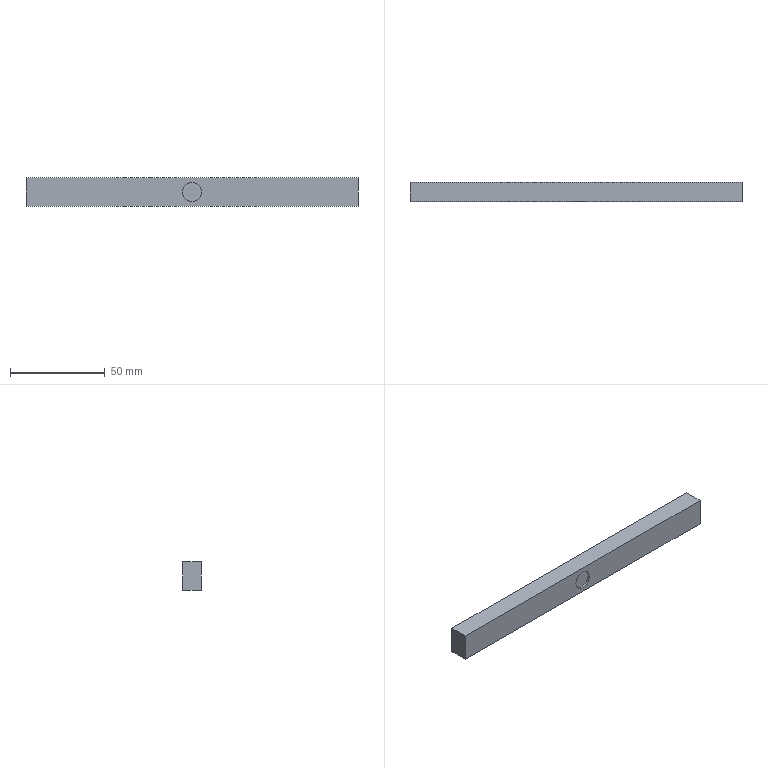Component | NX | MOTOR_ADJUST_PLATE | 1 solid | 8 faces | box 175 x 10 x 15 mm | volume 26171 mm3 | plane 7 | cylinder 1 | commonest cylinder face diameters 10 x1
STEP:
#1=CARTESIAN_POINT('',(0.,0.,0.));
#2=DIRECTION('',(0.,0.,1.));
#3=DIRECTION('',(1.,0.,0.));
#4=AXIS2_PLACEMENT_3D('',#1,#2,#3);
#5=CARTESIAN_POINT('',(955.989,728.423,123.5));
#6=VERTEX_POINT('',#5);
#7=CARTESIAN_POINT('',(955.989,728.423,138.5));
#8=VERTEX_POINT('',#7);
#9=CARTESIAN_POINT('',(955.989,728.423,123.5));
#10=DIRECTION('',(0.,0.,1.));
#11=VECTOR('',#10,1.);
#12=LINE('',#9,#11);
#13=CARTESIAN_POINT('',(955.989,738.423,123.5));
#14=DIRECTION('',(1.,0.,0.));
#15=DIRECTION('',(0.,0.,-1.));
#16=AXIS2_PLACEMENT_3D('',#13,#14,#15);
#17=PLANE('',#16);
#18=CARTESIAN_POINT('',(0.,-10.));
#19=DIRECTION('',(-1.,0.));
#20=VECTOR('',#19,1.);
#21=LINE('',#18,#20);
#22=(GEOMETRIC_REPRESENTATION_CONTEXT(2)PARAMETRIC_REPRESENTATION_CONTEXT()REPRESENTATION_CONTEXT('',''));
#23=DEFINITIONAL_REPRESENTATION('',(#21),#22);
#24=PCURVE('',#17,#23);
#25=CARTESIAN_POINT('',(0.,728.423,-15.));
#26=DIRECTION('',(0.,1.,0.));
#27=DIRECTION('',(0.,0.,1.));
#28=AXIS2_PLACEMENT_3D('',#25,#26,#27);
#29=PLANE('',#28);
#30=CARTESIAN_POINT('',(138.5,955.989));
#31=DIRECTION('',(1.,0.));
#32=VECTOR('',#31,1.);
#33=LINE('',#30,#32);
#34=(GEOMETRIC_REPRESENTATION_CONTEXT(2)PARAMETRIC_REPRESENTATION_CONTEXT()REPRESENTATION_CONTEXT('',''));
#35=DEFINITIONAL_REPRESENTATION('',(#33),#34);
#36=PCURVE('',#29,#35);
#37=SURFACE_CURVE('',#12,(#24,#36),.PCURVE_S1.);
#38=EDGE_CURVE('',#6,#8,#37,.T.);
#39=ORIENTED_EDGE('',*,*,#38,.T.);
#40=CARTESIAN_POINT('',(955.989,738.423,138.5));
#41=VERTEX_POINT('',#40);
#42=CARTESIAN_POINT('',(955.989,738.423,138.5));
#43=DIRECTION('',(0.,-1.,0.));
#44=VECTOR('',#43,1.);
#45=LINE('',#42,#44);
#46=CARTESIAN_POINT('',(-15.,0.));
#47=DIRECTION('',(0.,-1.));
#48=VECTOR('',#47,1.);
#49=LINE('',#46,#48);
#50=(GEOMETRIC_REPRESENTATION_CONTEXT(2)PARAMETRIC_REPRESENTATION_CONTEXT()REPRESENTATION_CONTEXT('',''));
#51=DEFINITIONAL_REPRESENTATION('',(#49),#50);
#52=PCURVE('',#17,#51);
#53=CARTESIAN_POINT('',(955.989,738.423,138.5));
#54=DIRECTION('',(0.,0.,-1.));
#55=DIRECTION('',(-1.,0.,0.));
#56=AXIS2_PLACEMENT_3D('',#53,#54,#55);
#57=PLANE('',#56);
#58=CARTESIAN_POINT('',(0.,0.));
#59=DIRECTION('',(0.,-1.));
#60=VECTOR('',#59,1.);
#61=LINE('',#58,#60);
#62=(GEOMETRIC_REPRESENTATION_CONTEXT(2)PARAMETRIC_REPRESENTATION_CONTEXT()REPRESENTATION_CONTEXT('',''));
#63=DEFINITIONAL_REPRESENTATION('',(#61),#62);
#64=PCURVE('',#57,#63);
#65=SURFACE_CURVE('',#45,(#52,#64),.PCURVE_S1.);
#66=EDGE_CURVE('',#41,#8,#65,.T.);
#67=ORIENTED_EDGE('',*,*,#66,.F.);
#68=CARTESIAN_POINT('',(955.989,738.423,123.5));
#69=VERTEX_POINT('',#68);
#70=CARTESIAN_POINT('',(955.989,738.423,123.5));
#71=DIRECTION('',(0.,0.,1.));
#72=VECTOR('',#71,1.);
#73=LINE('',#70,#72);
#74=CARTESIAN_POINT('',(0.,0.));
#75=DIRECTION('',(-1.,0.));
#76=VECTOR('',#75,1.);
#77=LINE('',#74,#76);
#78=(GEOMETRIC_REPRESENTATION_CONTEXT(2)PARAMETRIC_REPRESENTATION_CONTEXT()REPRESENTATION_CONTEXT('',''));
#79=DEFINITIONAL_REPRESENTATION('',(#77),#78);
#80=PCURVE('',#17,#79);
#81=CARTESIAN_POINT('',(0.,738.423,-15.));
#82=DIRECTION('',(0.,1.,0.));
#83=DIRECTION('',(0.,0.,1.));
#84=AXIS2_PLACEMENT_3D('',#81,#82,#83);
#85=PLANE('',#84);
#86=CARTESIAN_POINT('',(138.5,955.989));
#87=DIRECTION('',(1.,0.));
#88=VECTOR('',#87,1.);
#89=LINE('',#86,#88);
#90=(GEOMETRIC_REPRESENTATION_CONTEXT(2)PARAMETRIC_REPRESENTATION_CONTEXT()REPRESENTATION_CONTEXT('',''));
#91=DEFINITIONAL_REPRESENTATION('',(#89),#90);
#92=PCURVE('',#85,#91);
#93=SURFACE_CURVE('',#73,(#80,#92),.PCURVE_S1.);
#94=EDGE_CURVE('',#69,#41,#93,.T.);
#95=ORIENTED_EDGE('',*,*,#94,.F.);
#96=CARTESIAN_POINT('',(955.989,738.423,123.5));
#97=DIRECTION('',(0.,-1.,0.));
#98=VECTOR('',#97,1.);
#99=LINE('',#96,#98);
#100=CARTESIAN_POINT('',(0.,0.));
#101=DIRECTION('',(0.,-1.));
#102=VECTOR('',#101,1.);
#103=LINE('',#100,#102);
#104=(GEOMETRIC_REPRESENTATION_CONTEXT(2)PARAMETRIC_REPRESENTATION_CONTEXT()REPRESENTATION_CONTEXT('',''));
#105=DEFINITIONAL_REPRESENTATION('',(#103),#104);
#106=PCURVE('',#17,#105);
#107=CARTESIAN_POINT('',(1130.989,738.423,123.5));
#108=DIRECTION('',(-0.,0.,1.));
#109=DIRECTION('',(1.,0.,0.));
#110=AXIS2_PLACEMENT_3D('',#107,#108,#109);
#111=PLANE('',#110);
#112=CARTESIAN_POINT('',(-175.,0.));
#113=DIRECTION('',(0.,-1.));
#114=VECTOR('',#113,1.);
#115=LINE('',#112,#114);
#116=(GEOMETRIC_REPRESENTATION_CONTEXT(2)PARAMETRIC_REPRESENTATION_CONTEXT()REPRESENTATION_CONTEXT('',''));
#117=DEFINITIONAL_REPRESENTATION('',(#115),#116);
#118=PCURVE('',#111,#117);
#119=SURFACE_CURVE('',#99,(#106,#118),.PCURVE_S1.);
#120=EDGE_CURVE('',#69,#6,#119,.T.);
#121=ORIENTED_EDGE('',*,*,#120,.T.);
#122=EDGE_LOOP('',(#39,#67,#95,#121));
#123=FACE_BOUND('',#122,.T.);
#124=ADVANCED_FACE('',(#123),#17,.F.);
#125=CARTESIAN_POINT('',(1130.989,728.423,138.5));
#126=VERTEX_POINT('',#125);
#127=CARTESIAN_POINT('',(955.989,728.423,138.5));
#128=DIRECTION('',(1.,0.,0.));
#129=VECTOR('',#128,1.);
#130=LINE('',#127,#129);
#131=CARTESIAN_POINT('',(0.,-10.));
#132=DIRECTION('',(-1.,0.));
#133=VECTOR('',#132,1.);
#134=LINE('',#131,#133);
#135=(GEOMETRIC_REPRESENTATION_CONTEXT(2)PARAMETRIC_REPRESENTATION_CONTEXT()REPRESENTATION_CONTEXT('',''));
#136=DEFINITIONAL_REPRESENTATION('',(#134),#135);
#137=PCURVE('',#57,#136);
#138=CARTESIAN_POINT('',(153.5,955.989));
#139=DIRECTION('',(0.,1.));
#140=VECTOR('',#139,1.);
#141=LINE('',#138,#140);
#142=(GEOMETRIC_REPRESENTATION_CONTEXT(2)PARAMETRIC_REPRESENTATION_CONTEXT()REPRESENTATION_CONTEXT('',''));
#143=DEFINITIONAL_REPRESENTATION('',(#141),#142);
#144=PCURVE('',#29,#143);
#145=SURFACE_CURVE('',#130,(#137,#144),.PCURVE_S1.);
#146=EDGE_CURVE('',#8,#126,#145,.T.);
#147=ORIENTED_EDGE('',*,*,#146,.T.);
#148=CARTESIAN_POINT('',(1130.989,738.423,138.5));
#149=VERTEX_POINT('',#148);
#150=CARTESIAN_POINT('',(1130.989,738.423,138.5));
#151=DIRECTION('',(0.,-1.,0.));
#152=VECTOR('',#151,1.);
#153=LINE('',#150,#152);
#154=CARTESIAN_POINT('',(-175.,0.));
#155=DIRECTION('',(0.,-1.));
#156=VECTOR('',#155,1.);
#157=LINE('',#154,#156);
#158=(GEOMETRIC_REPRESENTATION_CONTEXT(2)PARAMETRIC_REPRESENTATION_CONTEXT()REPRESENTATION_CONTEXT('',''));
#159=DEFINITIONAL_REPRESENTATION('',(#157),#158);
#160=PCURVE('',#57,#159);
#161=CARTESIAN_POINT('',(1130.989,738.423,138.5));
#162=DIRECTION('',(-1.,0.,0.));
#163=DIRECTION('',(0.,0.,1.));
#164=AXIS2_PLACEMENT_3D('',#161,#162,#163);
#165=PLANE('',#164);
#166=CARTESIAN_POINT('',(0.,0.));
#167=DIRECTION('',(0.,-1.));
#168=VECTOR('',#167,1.);
#169=LINE('',#166,#168);
#170=(GEOMETRIC_REPRESENTATION_CONTEXT(2)PARAMETRIC_REPRESENTATION_CONTEXT()REPRESENTATION_CONTEXT('',''));
#171=DEFINITIONAL_REPRESENTATION('',(#169),#170);
#172=PCURVE('',#165,#171);
#173=SURFACE_CURVE('',#153,(#160,#172),.PCURVE_S1.);
#174=EDGE_CURVE('',#149,#126,#173,.T.);
#175=ORIENTED_EDGE('',*,*,#174,.F.);
#176=CARTESIAN_POINT('',(955.989,738.423,138.5));
#177=DIRECTION('',(1.,0.,0.));
#178=VECTOR('',#177,1.);
#179=LINE('',#176,#178);
#180=CARTESIAN_POINT('',(0.,0.));
#181=DIRECTION('',(-1.,0.));
#182=VECTOR('',#181,1.);
#183=LINE('',#180,#182);
#184=(GEOMETRIC_REPRESENTATION_CONTEXT(2)PARAMETRIC_REPRESENTATION_CONTEXT()REPRESENTATION_CONTEXT('',''));
#185=DEFINITIONAL_REPRESENTATION('',(#183),#184);
#186=PCURVE('',#57,#185);
#187=CARTESIAN_POINT('',(153.5,955.989));
#188=DIRECTION('',(0.,1.));
#189=VECTOR('',#188,1.);
#190=LINE('',#187,#189);
#191=(GEOMETRIC_REPRESENTATION_CONTEXT(2)PARAMETRIC_REPRESENTATION_CONTEXT()REPRESENTATION_CONTEXT('',''));
#192=DEFINITIONAL_REPRESENTATION('',(#190),#191);
#193=PCURVE('',#85,#192);
#194=SURFACE_CURVE('',#179,(#186,#193),.PCURVE_S1.);
#195=EDGE_CURVE('',#41,#149,#194,.T.);
#196=ORIENTED_EDGE('',*,*,#195,.F.);
#197=ORIENTED_EDGE('',*,*,#66,.T.);
#198=EDGE_LOOP('',(#147,#175,#196,#197));
#199=FACE_BOUND('',#198,.T.);
#200=ADVANCED_FACE('',(#199),#57,.F.);
#201=CARTESIAN_POINT('',(1130.989,728.423,123.5));
#202=VERTEX_POINT('',#201);
#203=CARTESIAN_POINT('',(1130.989,728.423,138.5));
#204=DIRECTION('',(0.,0.,-1.));
#205=VECTOR('',#204,1.);
#206=LINE('',#203,#205);
#207=CARTESIAN_POINT('',(0.,-10.));
#208=DIRECTION('',(-1.,0.));
#209=VECTOR('',#208,1.);
#210=LINE('',#207,#209);
#211=(GEOMETRIC_REPRESENTATION_CONTEXT(2)PARAMETRIC_REPRESENTATION_CONTEXT()REPRESENTATION_CONTEXT('',''));
#212=DEFINITIONAL_REPRESENTATION('',(#210),#211);
#213=PCURVE('',#165,#212);
#214=CARTESIAN_POINT('',(153.5,1130.989));
#215=DIRECTION('',(-1.,0.));
#216=VECTOR('',#215,1.);
#217=LINE('',#214,#216);
#218=(GEOMETRIC_REPRESENTATION_CONTEXT(2)PARAMETRIC_REPRESENTATION_CONTEXT()REPRESENTATION_CONTEXT('',''));
#219=DEFINITIONAL_REPRESENTATION('',(#217),#218);
#220=PCURVE('',#29,#219);
#221=SURFACE_CURVE('',#206,(#213,#220),.PCURVE_S1.);
#222=EDGE_CURVE('',#126,#202,#221,.T.);
#223=ORIENTED_EDGE('',*,*,#222,.T.);
#224=CARTESIAN_POINT('',(1130.989,738.423,123.5));
#225=VERTEX_POINT('',#224);
#226=CARTESIAN_POINT('',(1130.989,738.423,123.5));
#227=DIRECTION('',(0.,-1.,0.));
#228=VECTOR('',#227,1.);
#229=LINE('',#226,#228);
#230=CARTESIAN_POINT('',(-15.,0.));
#231=DIRECTION('',(0.,-1.));
#232=VECTOR('',#231,1.);
#233=LINE('',#230,#232);
#234=(GEOMETRIC_REPRESENTATION_CONTEXT(2)PARAMETRIC_REPRESENTATION_CONTEXT()REPRESENTATION_CONTEXT('',''));
#235=DEFINITIONAL_REPRESENTATION('',(#233),#234);
#236=PCURVE('',#165,#235);
#237=CARTESIAN_POINT('',(0.,0.));
#238=DIRECTION('',(0.,-1.));
#239=VECTOR('',#238,1.);
#240=LINE('',#237,#239);
#241=(GEOMETRIC_REPRESENTATION_CONTEXT(2)PARAMETRIC_REPRESENTATION_CONTEXT()REPRESENTATION_CONTEXT('',''));
#242=DEFINITIONAL_REPRESENTATION('',(#240),#241);
#243=PCURVE('',#111,#242);
#244=SURFACE_CURVE('',#229,(#236,#243),.PCURVE_S1.);
#245=EDGE_CURVE('',#225,#202,#244,.T.);
#246=ORIENTED_EDGE('',*,*,#245,.F.);
#247=CARTESIAN_POINT('',(1130.989,738.423,138.5));
#248=DIRECTION('',(0.,0.,-1.));
#249=VECTOR('',#248,1.);
#250=LINE('',#247,#249);
#251=CARTESIAN_POINT('',(0.,0.));
#252=DIRECTION('',(-1.,0.));
#253=VECTOR('',#252,1.);
#254=LINE('',#251,#253);
#255=(GEOMETRIC_REPRESENTATION_CONTEXT(2)PARAMETRIC_REPRESENTATION_CONTEXT()REPRESENTATION_CONTEXT('',''));
#256=DEFINITIONAL_REPRESENTATION('',(#254),#255);
#257=PCURVE('',#165,#256);
#258=CARTESIAN_POINT('',(153.5,1130.989));
#259=DIRECTION('',(-1.,0.));
#260=VECTOR('',#259,1.);
#261=LINE('',#258,#260);
#262=(GEOMETRIC_REPRESENTATION_CONTEXT(2)PARAMETRIC_REPRESENTATION_CONTEXT()REPRESENTATION_CONTEXT('',''));
#263=DEFINITIONAL_REPRESENTATION('',(#261),#262);
#264=PCURVE('',#85,#263);
#265=SURFACE_CURVE('',#250,(#257,#264),.PCURVE_S1.);
#266=EDGE_CURVE('',#149,#225,#265,.T.);
#267=ORIENTED_EDGE('',*,*,#266,.F.);
#268=ORIENTED_EDGE('',*,*,#174,.T.);
#269=EDGE_LOOP('',(#223,#246,#267,#268));
#270=FACE_BOUND('',#269,.T.);
#271=ADVANCED_FACE('',(#270),#165,.F.);
#272=CARTESIAN_POINT('',(1130.989,728.423,123.5));
#273=DIRECTION('',(-1.,0.,-0.));
#274=VECTOR('',#273,1.);
#275=LINE('',#272,#274);
#276=CARTESIAN_POINT('',(0.,-10.));
#277=DIRECTION('',(-1.,0.));
#278=VECTOR('',#277,1.);
#279=LINE('',#276,#278);
#280=(GEOMETRIC_REPRESENTATION_CONTEXT(2)PARAMETRIC_REPRESENTATION_CONTEXT()REPRESENTATION_CONTEXT('',''));
#281=DEFINITIONAL_REPRESENTATION('',(#279),#280);
#282=PCURVE('',#111,#281);
#283=CARTESIAN_POINT('',(138.5,1130.989));
#284=DIRECTION('',(-0.,-1.));
#285=VECTOR('',#284,1.);
#286=LINE('',#283,#285);
#287=(GEOMETRIC_REPRESENTATION_CONTEXT(2)PARAMETRIC_REPRESENTATION_CONTEXT()REPRESENTATION_CONTEXT('',''));
#288=DEFINITIONAL_REPRESENTATION('',(#286),#287);
#289=PCURVE('',#29,#288);
#290=SURFACE_CURVE('',#275,(#282,#289),.PCURVE_S1.);
#291=EDGE_CURVE('',#202,#6,#290,.T.);
#292=ORIENTED_EDGE('',*,*,#291,.T.);
#293=ORIENTED_EDGE('',*,*,#120,.F.);
#294=CARTESIAN_POINT('',(1130.989,738.423,123.5));
#295=DIRECTION('',(-1.,0.,-0.));
#296=VECTOR('',#295,1.);
#297=LINE('',#294,#296);
#298=CARTESIAN_POINT('',(0.,0.));
#299=DIRECTION('',(-1.,0.));
#300=VECTOR('',#299,1.);
#301=LINE('',#298,#300);
#302=(GEOMETRIC_REPRESENTATION_CONTEXT(2)PARAMETRIC_REPRESENTATION_CONTEXT()REPRESENTATION_CONTEXT('',''));
#303=DEFINITIONAL_REPRESENTATION('',(#301),#302);
#304=PCURVE('',#111,#303);
#305=CARTESIAN_POINT('',(138.5,1130.989));
#306=DIRECTION('',(-0.,-1.));
#307=VECTOR('',#306,1.);
#308=LINE('',#305,#307);
#309=(GEOMETRIC_REPRESENTATION_CONTEXT(2)PARAMETRIC_REPRESENTATION_CONTEXT()REPRESENTATION_CONTEXT('',''));
#310=DEFINITIONAL_REPRESENTATION('',(#308),#309);
#311=PCURVE('',#85,#310);
#312=SURFACE_CURVE('',#297,(#304,#311),.PCURVE_S1.);
#313=EDGE_CURVE('',#225,#69,#312,.T.);
#314=ORIENTED_EDGE('',*,*,#313,.F.);
#315=ORIENTED_EDGE('',*,*,#245,.T.);
#316=EDGE_LOOP('',(#292,#293,#314,#315));
#317=FACE_BOUND('',#316,.T.);
#318=ADVANCED_FACE('',(#317),#111,.F.);
#319=ORIENTED_EDGE('',*,*,#94,.T.);
#320=ORIENTED_EDGE('',*,*,#195,.T.);
#321=ORIENTED_EDGE('',*,*,#266,.T.);
#322=ORIENTED_EDGE('',*,*,#313,.T.);
#323=EDGE_LOOP('',(#319,#320,#321,#322));
#324=FACE_BOUND('',#323,.T.);
#325=ADVANCED_FACE('',(#324),#85,.T.);
#326=CARTESIAN_POINT('',(1048.489,728.423,131.));
#327=VERTEX_POINT('',#326);
#328=CARTESIAN_POINT('',(1043.489,728.423,131.));
#329=DIRECTION('',(0.,-1.,0.));
#330=DIRECTION('',(1.,0.,0.));
#331=AXIS2_PLACEMENT_3D('',#328,#329,#330);
#332=CIRCLE('',#331,5.);
#333=CARTESIAN_POINT('',(146.,1048.489));
#334=CARTESIAN_POINT('',(154.66,1048.489));
#335=CARTESIAN_POINT('',(150.33,1040.989));
#336=CARTESIAN_POINT('',(146.,1033.489));
#337=CARTESIAN_POINT('',(141.67,1040.989));
#338=CARTESIAN_POINT('',(137.34,1048.489));
#339=CARTESIAN_POINT('',(146.,1048.489));
#340=(BOUNDED_CURVE()B_SPLINE_CURVE(2,(#333,#334,#335,#336,#337,#338,#339),.UNSPECIFIED.,.T.,.F.)B_SPLINE_CURVE_WITH_KNOTS((1,2,2,2,2,1),(-2.094,0.,2.094,4.189,6.283,8.378),.UNSPECIFIED.)CURVE()GEOMETRIC_REPRESENTATION_ITEM()RATIONAL_B_SPLINE_CURVE((1.,0.5,1.,0.5,1.,0.5,1.))REPRESENTATION_ITEM(''));
#341=(GEOMETRIC_REPRESENTATION_CONTEXT(2)PARAMETRIC_REPRESENTATION_CONTEXT()REPRESENTATION_CONTEXT('',''));
#342=DEFINITIONAL_REPRESENTATION('',(#340),#341);
#343=PCURVE('',#29,#342);
#344=CARTESIAN_POINT('',(1043.489,729.423,131.));
#345=DIRECTION('',(0.,-1.,0.));
#346=DIRECTION('',(0.,0.,-1.));
#347=AXIS2_PLACEMENT_3D('',#344,#345,#346);
#348=CYLINDRICAL_SURFACE('',#347,5.);
#349=CARTESIAN_POINT('',(1.571,1.));
#350=DIRECTION('',(1.,0.));
#351=VECTOR('',#350,1.);
#352=LINE('',#349,#351);
#353=(GEOMETRIC_REPRESENTATION_CONTEXT(2)PARAMETRIC_REPRESENTATION_CONTEXT()REPRESENTATION_CONTEXT('',''));
#354=DEFINITIONAL_REPRESENTATION('',(#352),#353);
#355=PCURVE('',#348,#354);
#356=SURFACE_CURVE('',#332,(#343,#355),.PCURVE_S1.);
#357=EDGE_CURVE('',#327,#327,#356,.T.);
#358=ORIENTED_EDGE('',*,*,#357,.F.);
#359=EDGE_LOOP('',(#358));
#360=FACE_BOUND('',#359,.T.);
#361=ORIENTED_EDGE('',*,*,#38,.F.);
#362=ORIENTED_EDGE('',*,*,#291,.F.);
#363=ORIENTED_EDGE('',*,*,#222,.F.);
#364=ORIENTED_EDGE('',*,*,#146,.F.);
#365=EDGE_LOOP('',(#361,#362,#363,#364));
#366=FACE_BOUND('',#365,.T.);
#367=ADVANCED_FACE('',(#360,#366),#29,.F.);
#368=CARTESIAN_POINT('',(1048.489,729.423,131.));
#369=VERTEX_POINT('',#368);
#370=CARTESIAN_POINT('',(1043.489,729.423,131.));
#371=DIRECTION('',(0.,1.,0.));
#372=DIRECTION('',(1.,0.,0.));
#373=AXIS2_PLACEMENT_3D('',#370,#371,#372);
#374=CIRCLE('',#373,5.);
#375=CARTESIAN_POINT('',(7.854,0.));
#376=DIRECTION('',(-1.,0.));
#377=VECTOR('',#376,1.);
#378=LINE('',#375,#377);
#379=(GEOMETRIC_REPRESENTATION_CONTEXT(2)PARAMETRIC_REPRESENTATION_CONTEXT()REPRESENTATION_CONTEXT('',''));
#380=DEFINITIONAL_REPRESENTATION('',(#378),#379);
#381=PCURVE('',#348,#380);
#382=CARTESIAN_POINT('',(1043.489,729.423,131.));
#383=DIRECTION('',(0.,-1.,0.));
#384=DIRECTION('',(0.,0.,-1.));
#385=AXIS2_PLACEMENT_3D('',#382,#383,#384);
#386=PLANE('',#385);
#387=CARTESIAN_POINT('',(0.,5.));
#388=CARTESIAN_POINT('',(8.66,5.));
#389=CARTESIAN_POINT('',(4.33,-2.5));
#390=CARTESIAN_POINT('',(0.,-10.));
#391=CARTESIAN_POINT('',(-4.33,-2.5));
#392=CARTESIAN_POINT('',(-8.66,5.));
#393=CARTESIAN_POINT('',(0.,5.));
#394=(BOUNDED_CURVE()B_SPLINE_CURVE(2,(#387,#388,#389,#390,#391,#392,#393),.UNSPECIFIED.,.T.,.F.)B_SPLINE_CURVE_WITH_KNOTS((1,2,2,2,2,1),(-2.094,0.,2.094,4.189,6.283,8.378),.UNSPECIFIED.)CURVE()GEOMETRIC_REPRESENTATION_ITEM()RATIONAL_B_SPLINE_CURVE((1.,0.5,1.,0.5,1.,0.5,1.))REPRESENTATION_ITEM(''));
#395=(GEOMETRIC_REPRESENTATION_CONTEXT(2)PARAMETRIC_REPRESENTATION_CONTEXT()REPRESENTATION_CONTEXT('',''));
#396=DEFINITIONAL_REPRESENTATION('',(#394),#395);
#397=PCURVE('',#386,#396);
#398=SURFACE_CURVE('',#374,(#381,#397),.PCURVE_S1.);
#399=EDGE_CURVE('',#369,#369,#398,.T.);
#400=ORIENTED_EDGE('',*,*,#399,.F.);
#401=CARTESIAN_POINT('',(1048.489,729.423,131.));
#402=CARTESIAN_POINT('',(1048.489,728.423,131.));
#403=B_SPLINE_CURVE_WITH_KNOTS('',1,(#401,#402),.UNSPECIFIED.,.F.,.F.,(2,2),(0.,1.),.PIECEWISE_BEZIER_KNOTS.);
#404=CARTESIAN_POINT('',(7.854,0.));
#405=DIRECTION('',(0.,1.));
#406=VECTOR('',#405,1.);
#407=LINE('',#404,#406);
#408=(GEOMETRIC_REPRESENTATION_CONTEXT(2)PARAMETRIC_REPRESENTATION_CONTEXT()REPRESENTATION_CONTEXT('',''));
#409=DEFINITIONAL_REPRESENTATION('',(#407),#408);
#410=PCURVE('',#348,#409);
#411=CARTESIAN_POINT('',(1.571,0.));
#412=DIRECTION('',(0.,1.));
#413=VECTOR('',#412,1.);
#414=LINE('',#411,#413);
#415=(GEOMETRIC_REPRESENTATION_CONTEXT(2)PARAMETRIC_REPRESENTATION_CONTEXT()REPRESENTATION_CONTEXT('',''));
#416=DEFINITIONAL_REPRESENTATION('',(#414),#415);
#417=PCURVE('',#348,#416);
#418=SEAM_CURVE('',#403,(#410,#417),.PCURVE_S1.);
#419=EDGE_CURVE('',#369,#327,#418,.T.);
#420=ORIENTED_EDGE('',*,*,#419,.T.);
#421=ORIENTED_EDGE('',*,*,#357,.F.);
#422=ORIENTED_EDGE('',*,*,#419,.F.);
#423=EDGE_LOOP('',(#400,#420,#421,#422));
#424=FACE_BOUND('',#423,.F.);
#425=ADVANCED_FACE('',(#424),#348,.F.);
#426=ORIENTED_EDGE('',*,*,#399,.F.);
#427=EDGE_LOOP('',(#426));
#428=FACE_BOUND('',#427,.T.);
#429=ADVANCED_FACE('',(#428),#386,.T.);
#430=CLOSED_SHELL('',(#124,#200,#271,#318,#325,#367,#425,#429));
#431=MANIFOLD_SOLID_BREP('',#430);
#432=(LENGTH_UNIT()NAMED_UNIT(*)SI_UNIT(.MILLI.,.METRE.));
#433=UNCERTAINTY_MEASURE_WITH_UNIT(LENGTH_MEASURE(0.000002),#432,'','');
#434=(NAMED_UNIT(*)PLANE_ANGLE_UNIT()SI_UNIT($,.RADIAN.));
#435=(NAMED_UNIT(*)SI_UNIT($,.STERADIAN.)SOLID_ANGLE_UNIT());
#436=(GEOMETRIC_REPRESENTATION_CONTEXT(3)GLOBAL_UNCERTAINTY_ASSIGNED_CONTEXT((#433))GLOBAL_UNIT_ASSIGNED_CONTEXT((#432,#434,#435))REPRESENTATION_CONTEXT('',''));
#437=ADVANCED_BREP_SHAPE_REPRESENTATION('',(#4,#431),#436);